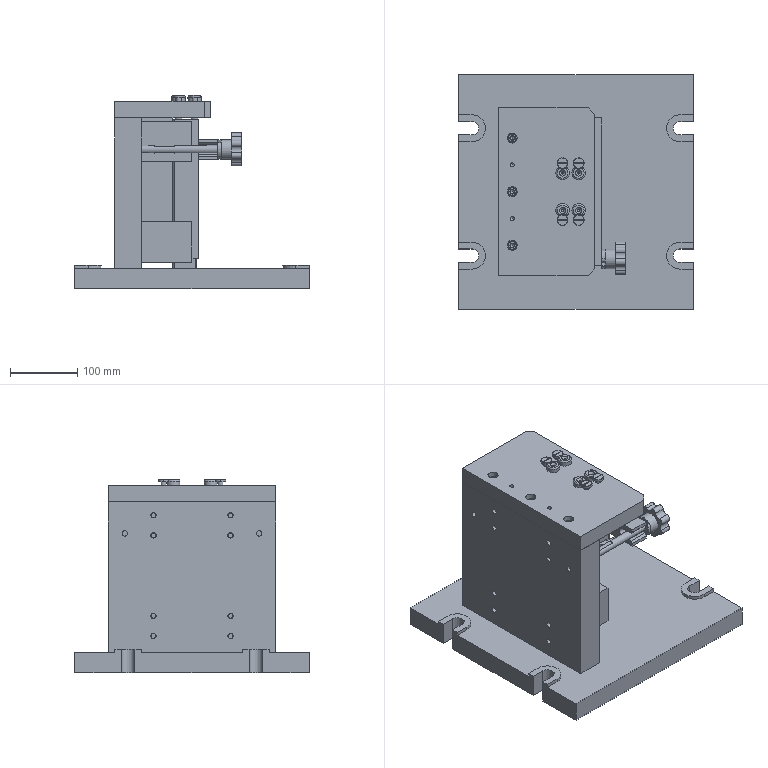Assembly | NX | mm | 35 component files | 35 solids | 804 faces | box 350 x 350 x 289 mm | volume 8393626 mm3 | plane 429 | cylinder 177 | cone 166 | torus 32 | commonest cylinder face diameters 8 x37 9 x14 15 x14 7.76 x14 13 x14 10 x11 20 x10 12 x10
Bill of materials:
unnamed part 1 | 1 |  | Solid knob-like body: a seven-lobed, star-shaped scalloped disc with a smaller plain cylindrical boss on one side, sharing the same axis.
unnamed part 2 | 4 |  | Slotted cheese-style headed pin or screw blank: a flat cylindrical head with one straight slot across it and a smooth cylindrical shank with a chamfered tip.
unnamed part 3 | 1 |  | Flat rectangular plate with two chamfered corners on one short edge and a pattern of through holes: a row of five holes along one long edge (alternating larger and smaller) and two clusters of four holes, each cluster with two sizes.
unnamed part 4 | 4 |  | Rectangular block with one chamfered (beveled) long edge and two parallel through holes running across its narrow dimension.
unnamed part 5 | 1 |  | Long flat bar with a clevis-like slot at each end: one end has an open slot with a rounded inner end and chamfered entry, and the other end has a square-bottomed slot. Small cross holes pass through the slotted end.
unnamed part 6 | 1 |  | Square flat plate with four open-ended U-slots on two opposite edges, each with a raised lip or boss around it. It has a central through hole and a line of five small holes in alternating sizes.
unnamed part 7 | 1 |  | Tall rectangular block with chamfered corners. It has a stepped side pocket or channel with curved (cylindrical) cutouts, a slot open at the bottom end, and several small holes on its faces and top.
unnamed part 8 | 4 |  | Headed pin or sleeve: a cylindrical head with a rounded top edge and a conical (countersunk) recess around a small central through hole, with a plain cylindrical shank. A small step or notch is cut into one side of the head.
unnamed part 9 | 1 |  | Flat open ring or C-shaped washer: an annular disc with a radial slot whose rounded inner end meets the central bore, making a keyhole-like opening.
unnamed part 10 | 1 |  | Stepped cylindrical shaft with three sections: a small-diameter end, a long medium-diameter body, and an enlarged end with two parallel flats and a transverse through hole.
unnamed part 11 | 1 |  | Thick block with a T-shaped profile: a main plate with a central raised rib. Countersunk or counterbored holes run in a row along the top face, and multiple through holes are spread over the large faces.
GB-T70.1-2000,M8x35 | 14 |  | Hexagon Socket Head Cap Screw, GB-T 70.1-2000,M8x35
unnamed part 12 | 1 |  | Long round shaft with a reduced-diameter end journal, a short collar shoulder next to it, and a shallow flat or relief section along part of the main body.
Mates:
1. concentric | support_plate_2 1 edge | fixture_base 1 edge
2. concentric | support_plate_2 1 edge | fixture_base 1 edge
3. concentric | support_plate 1 edge | support_plate_2 1 edge
4. concentric | support_plate 1 edge | support_plate_2 1 edge
5. concentric | block 4 edge | support_plate_2 1 edge
6. concentric | block 3 edge | support_plate_2 1 edge
7. fix | assembly component
8. bond | block 3 component | assembly component
9. bond | block 4 component | assembly component
10. bond | block 2 component | assembly component
11. bond | block 1 component | assembly component
12. linear | assembly datumaxis | assembly cartesiancoordinatesystem | assembly cartesiancoordinatesystem
13. linear | assembly datumaxis | assembly cartesiancoordinatesystem | assembly cartesiancoordinatesystem
14. concentric | drill_jig 4 edge | support_plate 1 edge
15. concentric | drill_jig 3 edge | support_plate 1 edge
16. concentric | drill_jig 2 edge | support_plate 1 edge
17. concentric | drill_jig 1 edge | support_plate 1 edge
18. parallel | drill_jig 4 face | support_plate 1 face
19. parallel | drill_jig 3 face | support_plate 1 face
20. parallel | drill_jig 2 face | support_plate 1 face
21. parallel | drill_jig 1 face | support_plate 1 face
22. touch align | drill_jig_screw 4 face | support_plate 1 face
23. touch align | drill_jig_screw 4 face | drill_jig 4 face
24. fix | assembly component
25. fix | assembly component
26. bond | drill_jig_screw 4 component | assembly component
27. bond | drill_jig_screw 3 component | assembly component
28. bond | drill_jig_screw 2 component | assembly component
29. bond | drill_jig_screw 1 component | assembly component
30. linear | assembly datumaxis | assembly datumaxis | assembly cartesiancoordinatesystem | assembly cartesiancoordinatesystem | assembly cartesiancoordinatesystem | assembly cartesiancoordinatesystem
31. touch align | product 1 face | drill_jig 1 face
32. touch align | product 1 face | block 4 face
33. touch align | product 1 face | support_plate_2 1 face
34. fix | fixture_base 1 component
35. concentric | locking_shaft 1 edge | support_plate_2 1 edge
36. concentric | locking_shaft_2 1 edge | support_plate_2 1 edge
37. parallel | locking_shaft_2 1 face | support_plate 1 face
38. concentric | clamp_plate 1 edge | locking_shaft_2 1 edge
39. parallel | clamp_plate 1 face | support_plate 1 face
40. touch align | washer 1 face | locking_shaft 1 face
41. touch align | washer 1 face | clamp_plate 1 face
42. concentric | thumb_nut 1 edge | washer 1 edge
43. fix | assembly component
44. bond | GB-T70_1-2000_M8x35 14 component | assembly component
45. bond | GB-T70_1-2000_M8x35 13 component | assembly component
46. linear | assembly datumaxis | assembly cartesiancoordinatesystem | assembly cartesiancoordinatesystem | assembly cartesiancoordinatesystem
47. bond | GB-T70_1-2000_M8x35 12 component | assembly component
48. concentric | GB-T70_1-2000_M8x35 11 edge | block 4 edge
49. concentric | GB-T70_1-2000_M8x35 10 edge | block 3 edge
50. concentric | GB-T70_1-2000_M8x35 9 edge | block 4 edge
51. concentric | GB-T70_1-2000_M8x35 8 edge | block 3 edge
52. concentric | GB-T70_1-2000_M8x35 7 edge | block 1 edge
53. concentric | GB-T70_1-2000_M8x35 6 edge | block 1 edge
54. concentric | GB-T70_1-2000_M8x35 5 edge | block 2 edge
55. concentric | GB-T70_1-2000_M8x35 4 edge | block 2 edge
56. concentric | GB-T70_1-2000_M8x35 3 edge | fixture_base 1 edge
57. fix | assembly component
58. bond | GB-T70_1-2000_M8x35 3 component | assembly component
59. bond | GB-T70_1-2000_M8x35 2 component | assembly component
60. bond | GB-T70_1-2000_M8x35 1 component | assembly component
61. linear | assembly datumaxis | assembly cartesiancoordinatesystem | assembly cartesiancoordinatesystem | assembly cartesiancoordinatesystem